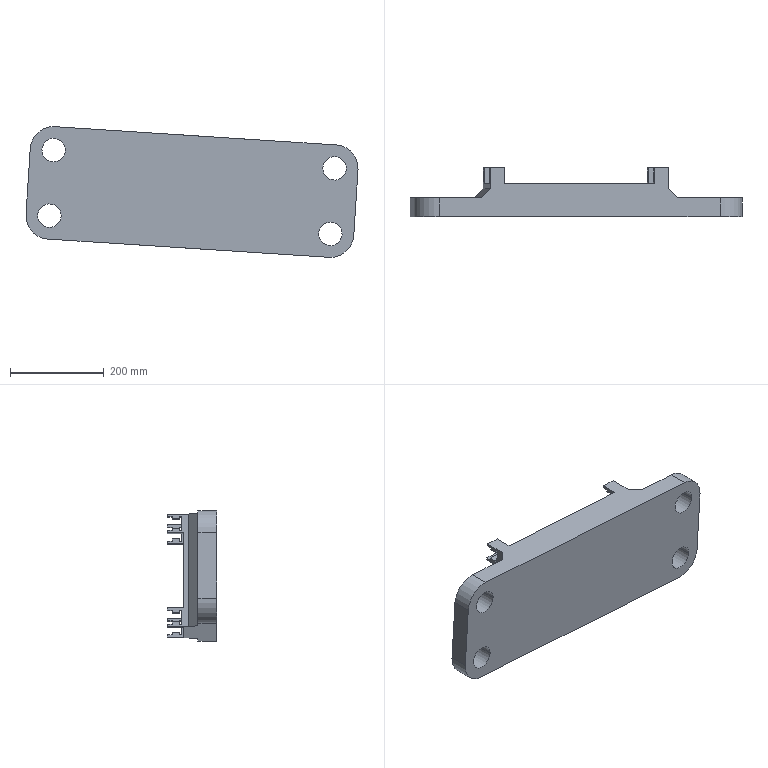Component | SolidWorks | X-AxisPedestal-1 | 1 solid | 84 faces | box 707.8 x 105 x 278.55 mm | volume 9228200 mm3 | plane 72 | cylinder 12 | commonest cylinder face diameters 50 x8 100 x4
build123d program:
from build123d import *

# Parameters (mm, degrees)
BOSS_EXTRUDE1_DEPTH   = 30
BOSS_EXTRUDE1_2_DEPTH = 30
LPATTERN1_COUNT       = 2
LPATTERN1_PITCH       = 350
SKETCH2_W             = 380
SKETCH2_H             = 240
BOSS_EXTRUDE2_DEPTH   = 30
SKETCH3_W             = 700
SKETCH3_H             = 240
BOSS_EXTRUDE3_DEPTH   = 40
CHAMFER1_SIZE         = 20
FILLET1_R             = 50
SKETCH5_R             = 25
CUT_EXTRUDE1_DEPTH    = 895.232


with BuildPart() as part:
    # Sketch1 → Boss-Extrude1 (new body)
    with BuildSketch(Plane.XY):
        Polygon((0, 470), (-10.5, 470), (-10.5, 474.5), (-25.5, 474.5), (-25.5, 470), (-30, 470), (-30, 500), (-25.5, 500), (-25.5, 495.5), (-10.5, 495.5), (-10.5, 500), (0, 500), (0, 505), (-35, 505), (-35, 465), (0, 465), align=None)
    boss_extrude1 = extrude(amount=-BOSS_EXTRUDE1_DEPTH)



with BuildPart() as body_2:
    # Sketch1 → Boss-Extrude1 2 (new body)
    with BuildSketch(Plane.XY):
        Polygon((0, 670), (-10.5, 670), (-10.5, 674.5), (-25.5, 674.5), (-25.5, 670), (-30, 670), (-30, 700), (-25.5, 700), (-25.5, 695.5), (-10.5, 695.5), (-10.5, 700), (0, 700), (0, 705), (-35, 705), (-35, 665), (0, 665), align=None)
    boss_extrude1_2 = extrude(amount=-BOSS_EXTRUDE1_2_DEPTH)


with BuildPart() as lpattern1_1:
    # LPattern1: pattern copy
    add(boss_extrude1.moved(Location(Vector(0, 0, -1) * (1 * LPATTERN1_PITCH))))


with BuildPart() as lpattern1_2:
    # LPattern1: pattern copy
    add(boss_extrude1_2.moved(Location(Vector(0, 0, -1) * (1 * LPATTERN1_PITCH))))


with BuildPart() as part_1:
    add(part.part)

    add(body_2.part)  # Boss-Extrude2 merges body 2

    add(lpattern1_1.part)  # Boss-Extrude2 merges LPattern1_1

    add(lpattern1_2.part)  # Boss-Extrude2 merges LPattern1_2
    # Sketch2 → Boss-Extrude2 (add)
    with BuildSketch(Plane.ZY.offset(35)):
        with Locations((-190, 585)):
            Rectangle(SKETCH2_W, SKETCH2_H)
    extrude(amount=BOSS_EXTRUDE2_DEPTH)

    # Sketch3 → Boss-Extrude3 (add)
    with BuildSketch(Plane.ZY.offset(65)):
        with Locations((-190, 585)):
            Rectangle(SKETCH3_W, SKETCH3_H)
    extrude(amount=BOSS_EXTRUDE3_DEPTH)

    # Chamfer1
    chamfer1_edges = [part_1.edges().sort_by_distance(p)[0] for p in [
        (-65, 585, -380),
        (-65, 585, 0),
    ]]
    chamfer(chamfer1_edges, length=CHAMFER1_SIZE)

    # Fillet1
    fillet1_edges = [part_1.edges().sort_by_distance(p)[0] for p in [
        (-85, 465, 160),
        (-85, 705, 160),
        (-85, 705, -540),
        (-85, 465, -540),
    ]]
    fillet(fillet1_edges, radius=FILLET1_R)

    # Sketch5 → Cut-Extrude1 (cut, through all)
    with BuildSketch(Plane.ZY.offset(105)):
        with Locations((110, 655)):
            Circle(SKETCH5_R)
        with Locations((110, 515)):
            Circle(SKETCH5_R)
        with Locations((-490, 515)):
            Circle(SKETCH5_R)
        with Locations((-490, 655)):
            Circle(SKETCH5_R)
    extrude(amount=-CUT_EXTRUDE1_DEPTH, mode=Mode.SUBTRACT)


solid = part_1.part

# Placed as in the assembly
solid = solid.moved(Location((136.66, -696, -884.937), (180, 86.288, -90)))